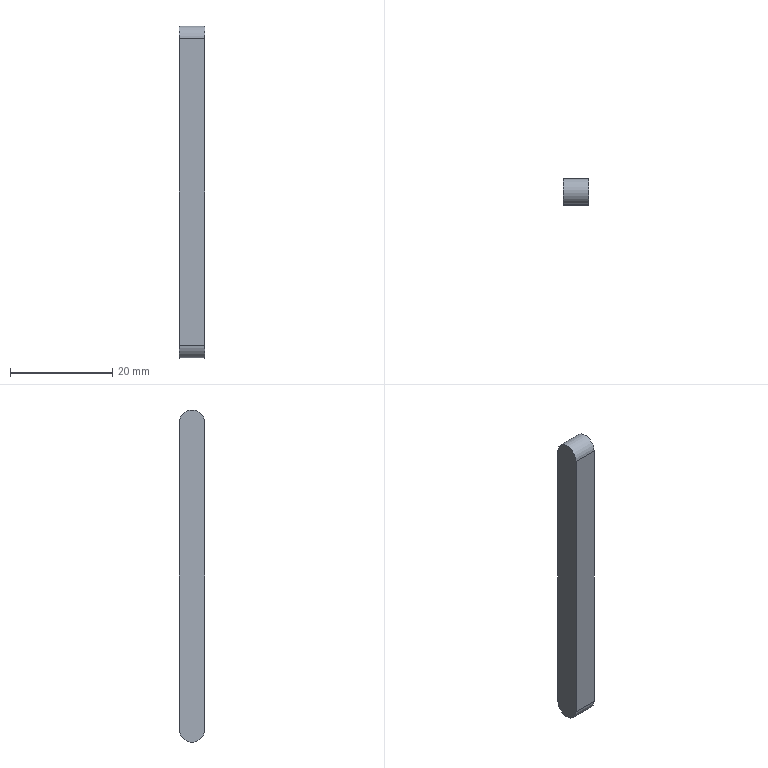Component | NX | KEY | 1 solid | 6 faces | box 5 x 5 x 65 mm | volume 1598 mm3 | plane 4 | cylinder 2 | commonest cylinder face diameters 5 x2
STEP:
#1=CARTESIAN_POINT('',(0.,0.,0.));
#2=DIRECTION('',(0.,0.,1.));
#3=DIRECTION('',(1.,0.,0.));
#4=AXIS2_PLACEMENT_3D('',#1,#2,#3);
#5=CARTESIAN_POINT('',(12.5,-2.5,145.));
#6=VERTEX_POINT('',#5);
#7=CARTESIAN_POINT('',(12.5,-2.5,205.));
#8=VERTEX_POINT('',#7);
#9=CARTESIAN_POINT('',(12.5,-2.5,175.));
#10=DIRECTION('',(0.,0.,1.));
#11=VECTOR('',#10,1.);
#12=LINE('',#9,#11);
#13=CARTESIAN_POINT('',(12.5,-0.,175.));
#14=DIRECTION('',(1.,0.,0.));
#15=DIRECTION('',(0.,0.,-1.));
#16=AXIS2_PLACEMENT_3D('',#13,#14,#15);
#17=PLANE('',#16);
#18=CARTESIAN_POINT('',(0.,-2.5));
#19=DIRECTION('',(-1.,0.));
#20=VECTOR('',#19,1.);
#21=LINE('',#18,#20);
#22=(GEOMETRIC_REPRESENTATION_CONTEXT(2)PARAMETRIC_REPRESENTATION_CONTEXT()REPRESENTATION_CONTEXT('',''));
#23=DEFINITIONAL_REPRESENTATION('',(#21),#22);
#24=PCURVE('',#17,#23);
#25=CARTESIAN_POINT('',(7.5,-2.5,175.));
#26=DIRECTION('',(0.,-1.,0.));
#27=DIRECTION('',(-1.,0.,0.));
#28=AXIS2_PLACEMENT_3D('',#25,#26,#27);
#29=PLANE('',#28);
#30=CARTESIAN_POINT('',(-5.,0.));
#31=DIRECTION('',(0.,-1.));
#32=VECTOR('',#31,1.);
#33=LINE('',#30,#32);
#34=(GEOMETRIC_REPRESENTATION_CONTEXT(2)PARAMETRIC_REPRESENTATION_CONTEXT()REPRESENTATION_CONTEXT('',''));
#35=DEFINITIONAL_REPRESENTATION('',(#33),#34);
#36=PCURVE('',#29,#35);
#37=SURFACE_CURVE('',#12,(#24,#36),.PCURVE_S1.);
#38=EDGE_CURVE('',#6,#8,#37,.T.);
#39=ORIENTED_EDGE('',*,*,#38,.F.);
#40=CARTESIAN_POINT('',(12.5,2.5,145.));
#41=VERTEX_POINT('',#40);
#42=CARTESIAN_POINT('',(12.5,-0.,145.));
#43=DIRECTION('',(1.,0.,0.));
#44=DIRECTION('',(0.,0.,-1.));
#45=AXIS2_PLACEMENT_3D('',#42,#43,#44);
#46=CIRCLE('',#45,2.5);
#47=CARTESIAN_POINT('',(30.,0.));
#48=DIRECTION('',(1.,0.));
#49=AXIS2_PLACEMENT_2D('',#47,#48);
#50=CIRCLE('',#49,2.5);
#51=(GEOMETRIC_REPRESENTATION_CONTEXT(2)PARAMETRIC_REPRESENTATION_CONTEXT()REPRESENTATION_CONTEXT('',''));
#52=DEFINITIONAL_REPRESENTATION('',(#50),#51);
#53=PCURVE('',#17,#52);
#54=CARTESIAN_POINT('',(7.5,-0.,145.));
#55=DIRECTION('',(1.,0.,0.));
#56=DIRECTION('',(0.,0.,-1.));
#57=AXIS2_PLACEMENT_3D('',#54,#55,#56);
#58=CYLINDRICAL_SURFACE('',#57,2.5);
#59=CARTESIAN_POINT('',(0.,5.));
#60=DIRECTION('',(1.,0.));
#61=VECTOR('',#60,1.);
#62=LINE('',#59,#61);
#63=(GEOMETRIC_REPRESENTATION_CONTEXT(2)PARAMETRIC_REPRESENTATION_CONTEXT()REPRESENTATION_CONTEXT('',''));
#64=DEFINITIONAL_REPRESENTATION('',(#62),#63);
#65=PCURVE('',#58,#64);
#66=SURFACE_CURVE('',#46,(#53,#65),.PCURVE_S1.);
#67=EDGE_CURVE('',#6,#41,#66,.T.);
#68=ORIENTED_EDGE('',*,*,#67,.T.);
#69=CARTESIAN_POINT('',(12.5,2.5,205.));
#70=VERTEX_POINT('',#69);
#71=CARTESIAN_POINT('',(12.5,2.5,175.));
#72=DIRECTION('',(0.,0.,-1.));
#73=VECTOR('',#72,1.);
#74=LINE('',#71,#73);
#75=CARTESIAN_POINT('',(0.,2.5));
#76=DIRECTION('',(1.,0.));
#77=VECTOR('',#76,1.);
#78=LINE('',#75,#77);
#79=(GEOMETRIC_REPRESENTATION_CONTEXT(2)PARAMETRIC_REPRESENTATION_CONTEXT()REPRESENTATION_CONTEXT('',''));
#80=DEFINITIONAL_REPRESENTATION('',(#78),#79);
#81=PCURVE('',#17,#80);
#82=CARTESIAN_POINT('',(7.5,2.5,175.));
#83=DIRECTION('',(0.,1.,0.));
#84=DIRECTION('',(1.,0.,0.));
#85=AXIS2_PLACEMENT_3D('',#82,#83,#84);
#86=PLANE('',#85);
#87=CARTESIAN_POINT('',(5.,0.));
#88=DIRECTION('',(0.,1.));
#89=VECTOR('',#88,1.);
#90=LINE('',#87,#89);
#91=(GEOMETRIC_REPRESENTATION_CONTEXT(2)PARAMETRIC_REPRESENTATION_CONTEXT()REPRESENTATION_CONTEXT('',''));
#92=DEFINITIONAL_REPRESENTATION('',(#90),#91);
#93=PCURVE('',#86,#92);
#94=SURFACE_CURVE('',#74,(#81,#93),.PCURVE_S1.);
#95=EDGE_CURVE('',#70,#41,#94,.T.);
#96=ORIENTED_EDGE('',*,*,#95,.F.);
#97=CARTESIAN_POINT('',(12.5,-0.,205.));
#98=DIRECTION('',(1.,0.,0.));
#99=DIRECTION('',(0.,0.,-1.));
#100=AXIS2_PLACEMENT_3D('',#97,#98,#99);
#101=CIRCLE('',#100,2.5);
#102=CARTESIAN_POINT('',(-30.,0.));
#103=DIRECTION('',(1.,0.));
#104=AXIS2_PLACEMENT_2D('',#102,#103);
#105=CIRCLE('',#104,2.5);
#106=(GEOMETRIC_REPRESENTATION_CONTEXT(2)PARAMETRIC_REPRESENTATION_CONTEXT()REPRESENTATION_CONTEXT('',''));
#107=DEFINITIONAL_REPRESENTATION('',(#105),#106);
#108=PCURVE('',#17,#107);
#109=CARTESIAN_POINT('',(7.5,-0.,205.));
#110=DIRECTION('',(1.,0.,0.));
#111=DIRECTION('',(0.,0.,-1.));
#112=AXIS2_PLACEMENT_3D('',#109,#110,#111);
#113=CYLINDRICAL_SURFACE('',#112,2.5);
#114=CARTESIAN_POINT('',(0.,5.));
#115=DIRECTION('',(1.,0.));
#116=VECTOR('',#115,1.);
#117=LINE('',#114,#116);
#118=(GEOMETRIC_REPRESENTATION_CONTEXT(2)PARAMETRIC_REPRESENTATION_CONTEXT()REPRESENTATION_CONTEXT('',''));
#119=DEFINITIONAL_REPRESENTATION('',(#117),#118);
#120=PCURVE('',#113,#119);
#121=SURFACE_CURVE('',#101,(#108,#120),.PCURVE_S1.);
#122=EDGE_CURVE('',#70,#8,#121,.T.);
#123=ORIENTED_EDGE('',*,*,#122,.T.);
#124=EDGE_LOOP('',(#39,#68,#96,#123));
#125=FACE_BOUND('',#124,.T.);
#126=ADVANCED_FACE('',(#125),#17,.T.);
#127=CARTESIAN_POINT('',(7.5,-2.5,205.));
#128=VERTEX_POINT('',#127);
#129=CARTESIAN_POINT('',(7.5,-2.5,145.));
#130=VERTEX_POINT('',#129);
#131=CARTESIAN_POINT('',(7.5,-2.5,175.));
#132=DIRECTION('',(0.,0.,-1.));
#133=VECTOR('',#132,1.);
#134=LINE('',#131,#133);
#135=CARTESIAN_POINT('',(0.,0.));
#136=DIRECTION('',(0.,1.));
#137=VECTOR('',#136,1.);
#138=LINE('',#135,#137);
#139=(GEOMETRIC_REPRESENTATION_CONTEXT(2)PARAMETRIC_REPRESENTATION_CONTEXT()REPRESENTATION_CONTEXT('',''));
#140=DEFINITIONAL_REPRESENTATION('',(#138),#139);
#141=PCURVE('',#29,#140);
#142=CARTESIAN_POINT('',(7.5,-0.,175.));
#143=DIRECTION('',(-1.,0.,0.));
#144=DIRECTION('',(0.,0.,1.));
#145=AXIS2_PLACEMENT_3D('',#142,#143,#144);
#146=PLANE('',#145);
#147=CARTESIAN_POINT('',(0.,-2.5));
#148=DIRECTION('',(-1.,0.));
#149=VECTOR('',#148,1.);
#150=LINE('',#147,#149);
#151=(GEOMETRIC_REPRESENTATION_CONTEXT(2)PARAMETRIC_REPRESENTATION_CONTEXT()REPRESENTATION_CONTEXT('',''));
#152=DEFINITIONAL_REPRESENTATION('',(#150),#151);
#153=PCURVE('',#146,#152);
#154=SURFACE_CURVE('',#134,(#141,#153),.PCURVE_S1.);
#155=EDGE_CURVE('',#128,#130,#154,.T.);
#156=ORIENTED_EDGE('',*,*,#155,.T.);
#157=CARTESIAN_POINT('',(7.5,-2.5,145.));
#158=DIRECTION('',(1.,0.,0.));
#159=VECTOR('',#158,1.);
#160=LINE('',#157,#159);
#161=CARTESIAN_POINT('',(0.,30.));
#162=DIRECTION('',(-1.,0.));
#163=VECTOR('',#162,1.);
#164=LINE('',#161,#163);
#165=(GEOMETRIC_REPRESENTATION_CONTEXT(2)PARAMETRIC_REPRESENTATION_CONTEXT()REPRESENTATION_CONTEXT('',''));
#166=DEFINITIONAL_REPRESENTATION('',(#164),#165);
#167=PCURVE('',#29,#166);
#168=CARTESIAN_POINT('',(4.712,0.));
#169=DIRECTION('',(0.,1.));
#170=VECTOR('',#169,1.);
#171=LINE('',#168,#170);
#172=(GEOMETRIC_REPRESENTATION_CONTEXT(2)PARAMETRIC_REPRESENTATION_CONTEXT()REPRESENTATION_CONTEXT('',''));
#173=DEFINITIONAL_REPRESENTATION('',(#171),#172);
#174=PCURVE('',#58,#173);
#175=SURFACE_CURVE('',#160,(#167,#174),.PCURVE_S1.);
#176=EDGE_CURVE('',#130,#6,#175,.T.);
#177=ORIENTED_EDGE('',*,*,#176,.T.);
#178=ORIENTED_EDGE('',*,*,#38,.T.);
#179=CARTESIAN_POINT('',(7.5,-2.5,205.));
#180=DIRECTION('',(-1.,0.,0.));
#181=VECTOR('',#180,1.);
#182=LINE('',#179,#181);
#183=CARTESIAN_POINT('',(0.,-30.));
#184=DIRECTION('',(1.,0.));
#185=VECTOR('',#184,1.);
#186=LINE('',#183,#185);
#187=(GEOMETRIC_REPRESENTATION_CONTEXT(2)PARAMETRIC_REPRESENTATION_CONTEXT()REPRESENTATION_CONTEXT('',''));
#188=DEFINITIONAL_REPRESENTATION('',(#186),#187);
#189=PCURVE('',#29,#188);
#190=CARTESIAN_POINT('',(4.712,0.));
#191=DIRECTION('',(0.,-1.));
#192=VECTOR('',#191,1.);
#193=LINE('',#190,#192);
#194=(GEOMETRIC_REPRESENTATION_CONTEXT(2)PARAMETRIC_REPRESENTATION_CONTEXT()REPRESENTATION_CONTEXT('',''));
#195=DEFINITIONAL_REPRESENTATION('',(#193),#194);
#196=PCURVE('',#113,#195);
#197=SURFACE_CURVE('',#182,(#189,#196),.PCURVE_S1.);
#198=EDGE_CURVE('',#8,#128,#197,.T.);
#199=ORIENTED_EDGE('',*,*,#198,.T.);
#200=EDGE_LOOP('',(#156,#177,#178,#199));
#201=FACE_BOUND('',#200,.T.);
#202=ADVANCED_FACE('',(#201),#29,.T.);
#203=ORIENTED_EDGE('',*,*,#95,.T.);
#204=CARTESIAN_POINT('',(7.5,2.5,145.));
#205=VERTEX_POINT('',#204);
#206=CARTESIAN_POINT('',(7.5,2.5,145.));
#207=DIRECTION('',(-1.,0.,0.));
#208=VECTOR('',#207,1.);
#209=LINE('',#206,#208);
#210=CARTESIAN_POINT('',(0.,30.));
#211=DIRECTION('',(-1.,0.));
#212=VECTOR('',#211,1.);
#213=LINE('',#210,#212);
#214=(GEOMETRIC_REPRESENTATION_CONTEXT(2)PARAMETRIC_REPRESENTATION_CONTEXT()REPRESENTATION_CONTEXT('',''));
#215=DEFINITIONAL_REPRESENTATION('',(#213),#214);
#216=PCURVE('',#86,#215);
#217=CARTESIAN_POINT('',(7.854,0.));
#218=DIRECTION('',(0.,-1.));
#219=VECTOR('',#218,1.);
#220=LINE('',#217,#219);
#221=(GEOMETRIC_REPRESENTATION_CONTEXT(2)PARAMETRIC_REPRESENTATION_CONTEXT()REPRESENTATION_CONTEXT('',''));
#222=DEFINITIONAL_REPRESENTATION('',(#220),#221);
#223=PCURVE('',#58,#222);
#224=SURFACE_CURVE('',#209,(#216,#223),.PCURVE_S1.);
#225=EDGE_CURVE('',#41,#205,#224,.T.);
#226=ORIENTED_EDGE('',*,*,#225,.T.);
#227=CARTESIAN_POINT('',(7.5,2.5,205.));
#228=VERTEX_POINT('',#227);
#229=CARTESIAN_POINT('',(7.5,2.5,175.));
#230=DIRECTION('',(0.,0.,1.));
#231=VECTOR('',#230,1.);
#232=LINE('',#229,#231);
#233=CARTESIAN_POINT('',(0.,0.));
#234=DIRECTION('',(0.,-1.));
#235=VECTOR('',#234,1.);
#236=LINE('',#233,#235);
#237=(GEOMETRIC_REPRESENTATION_CONTEXT(2)PARAMETRIC_REPRESENTATION_CONTEXT()REPRESENTATION_CONTEXT('',''));
#238=DEFINITIONAL_REPRESENTATION('',(#236),#237);
#239=PCURVE('',#86,#238);
#240=CARTESIAN_POINT('',(0.,2.5));
#241=DIRECTION('',(1.,0.));
#242=VECTOR('',#241,1.);
#243=LINE('',#240,#242);
#244=(GEOMETRIC_REPRESENTATION_CONTEXT(2)PARAMETRIC_REPRESENTATION_CONTEXT()REPRESENTATION_CONTEXT('',''));
#245=DEFINITIONAL_REPRESENTATION('',(#243),#244);
#246=PCURVE('',#146,#245);
#247=SURFACE_CURVE('',#232,(#239,#246),.PCURVE_S1.);
#248=EDGE_CURVE('',#205,#228,#247,.T.);
#249=ORIENTED_EDGE('',*,*,#248,.T.);
#250=CARTESIAN_POINT('',(7.5,2.5,205.));
#251=DIRECTION('',(1.,0.,0.));
#252=VECTOR('',#251,1.);
#253=LINE('',#250,#252);
#254=CARTESIAN_POINT('',(0.,-30.));
#255=DIRECTION('',(1.,0.));
#256=VECTOR('',#255,1.);
#257=LINE('',#254,#256);
#258=(GEOMETRIC_REPRESENTATION_CONTEXT(2)PARAMETRIC_REPRESENTATION_CONTEXT()REPRESENTATION_CONTEXT('',''));
#259=DEFINITIONAL_REPRESENTATION('',(#257),#258);
#260=PCURVE('',#86,#259);
#261=CARTESIAN_POINT('',(1.571,0.));
#262=DIRECTION('',(0.,1.));
#263=VECTOR('',#262,1.);
#264=LINE('',#261,#263);
#265=(GEOMETRIC_REPRESENTATION_CONTEXT(2)PARAMETRIC_REPRESENTATION_CONTEXT()REPRESENTATION_CONTEXT('',''));
#266=DEFINITIONAL_REPRESENTATION('',(#264),#265);
#267=PCURVE('',#113,#266);
#268=SURFACE_CURVE('',#253,(#260,#267),.PCURVE_S1.);
#269=EDGE_CURVE('',#228,#70,#268,.T.);
#270=ORIENTED_EDGE('',*,*,#269,.T.);
#271=EDGE_LOOP('',(#203,#226,#249,#270));
#272=FACE_BOUND('',#271,.T.);
#273=ADVANCED_FACE('',(#272),#86,.T.);
#274=CARTESIAN_POINT('',(7.5,-0.,145.));
#275=DIRECTION('',(-1.,0.,0.));
#276=DIRECTION('',(0.,0.,1.));
#277=AXIS2_PLACEMENT_3D('',#274,#275,#276);
#278=CIRCLE('',#277,2.5);
#279=CARTESIAN_POINT('',(-30.,0.));
#280=DIRECTION('',(1.,0.));
#281=AXIS2_PLACEMENT_2D('',#279,#280);
#282=CIRCLE('',#281,2.5);
#283=(GEOMETRIC_REPRESENTATION_CONTEXT(2)PARAMETRIC_REPRESENTATION_CONTEXT()REPRESENTATION_CONTEXT('',''));
#284=DEFINITIONAL_REPRESENTATION('',(#282),#283);
#285=PCURVE('',#146,#284);
#286=CARTESIAN_POINT('',(9.425,0.));
#287=DIRECTION('',(-1.,0.));
#288=VECTOR('',#287,1.);
#289=LINE('',#286,#288);
#290=(GEOMETRIC_REPRESENTATION_CONTEXT(2)PARAMETRIC_REPRESENTATION_CONTEXT()REPRESENTATION_CONTEXT('',''));
#291=DEFINITIONAL_REPRESENTATION('',(#289),#290);
#292=PCURVE('',#58,#291);
#293=SURFACE_CURVE('',#278,(#285,#292),.PCURVE_S1.);
#294=EDGE_CURVE('',#205,#130,#293,.T.);
#295=ORIENTED_EDGE('',*,*,#294,.T.);
#296=ORIENTED_EDGE('',*,*,#155,.F.);
#297=CARTESIAN_POINT('',(7.5,-0.,205.));
#298=DIRECTION('',(-1.,0.,0.));
#299=DIRECTION('',(0.,0.,1.));
#300=AXIS2_PLACEMENT_3D('',#297,#298,#299);
#301=CIRCLE('',#300,2.5);
#302=CARTESIAN_POINT('',(30.,0.));
#303=DIRECTION('',(1.,0.));
#304=AXIS2_PLACEMENT_2D('',#302,#303);
#305=CIRCLE('',#304,2.5);
#306=(GEOMETRIC_REPRESENTATION_CONTEXT(2)PARAMETRIC_REPRESENTATION_CONTEXT()REPRESENTATION_CONTEXT('',''));
#307=DEFINITIONAL_REPRESENTATION('',(#305),#306);
#308=PCURVE('',#146,#307);
#309=CARTESIAN_POINT('',(9.425,0.));
#310=DIRECTION('',(-1.,0.));
#311=VECTOR('',#310,1.);
#312=LINE('',#309,#311);
#313=(GEOMETRIC_REPRESENTATION_CONTEXT(2)PARAMETRIC_REPRESENTATION_CONTEXT()REPRESENTATION_CONTEXT('',''));
#314=DEFINITIONAL_REPRESENTATION('',(#312),#313);
#315=PCURVE('',#113,#314);
#316=SURFACE_CURVE('',#301,(#308,#315),.PCURVE_S1.);
#317=EDGE_CURVE('',#128,#228,#316,.T.);
#318=ORIENTED_EDGE('',*,*,#317,.T.);
#319=ORIENTED_EDGE('',*,*,#248,.F.);
#320=EDGE_LOOP('',(#295,#296,#318,#319));
#321=FACE_BOUND('',#320,.T.);
#322=ADVANCED_FACE('',(#321),#146,.T.);
#323=ORIENTED_EDGE('',*,*,#67,.F.);
#324=ORIENTED_EDGE('',*,*,#176,.F.);
#325=ORIENTED_EDGE('',*,*,#294,.F.);
#326=ORIENTED_EDGE('',*,*,#225,.F.);
#327=EDGE_LOOP('',(#323,#324,#325,#326));
#328=FACE_BOUND('',#327,.T.);
#329=ADVANCED_FACE('',(#328),#58,.T.);
#330=ORIENTED_EDGE('',*,*,#122,.F.);
#331=ORIENTED_EDGE('',*,*,#269,.F.);
#332=ORIENTED_EDGE('',*,*,#317,.F.);
#333=ORIENTED_EDGE('',*,*,#198,.F.);
#334=EDGE_LOOP('',(#330,#331,#332,#333));
#335=FACE_BOUND('',#334,.T.);
#336=ADVANCED_FACE('',(#335),#113,.T.);
#337=CLOSED_SHELL('',(#126,#202,#273,#322,#329,#336));
#338=MANIFOLD_SOLID_BREP('',#337);
#339=(LENGTH_UNIT()NAMED_UNIT(*)SI_UNIT(.MILLI.,.METRE.));
#340=UNCERTAINTY_MEASURE_WITH_UNIT(LENGTH_MEASURE(0.0000001),#339,'','');
#341=(NAMED_UNIT(*)PLANE_ANGLE_UNIT()SI_UNIT($,.RADIAN.));
#342=(NAMED_UNIT(*)SI_UNIT($,.STERADIAN.)SOLID_ANGLE_UNIT());
#343=(GEOMETRIC_REPRESENTATION_CONTEXT(3)GLOBAL_UNCERTAINTY_ASSIGNED_CONTEXT((#340))GLOBAL_UNIT_ASSIGNED_CONTEXT((#339,#341,#342))REPRESENTATION_CONTEXT('',''));
#344=ADVANCED_BREP_SHAPE_REPRESENTATION('',(#4,#338),#343);